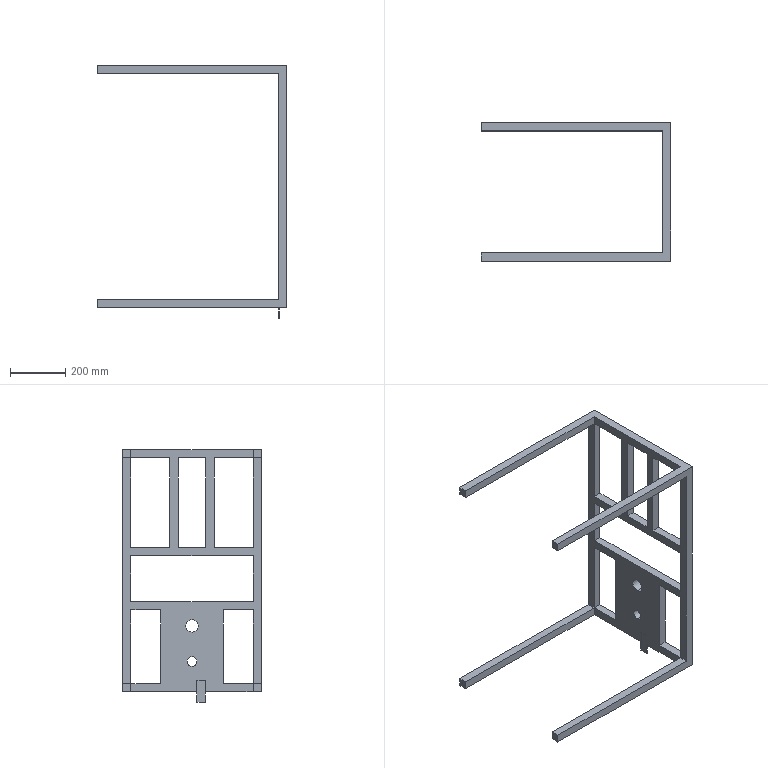Component | SolidWorks | Frame-1 | 1 solid | 55 faces | volume 7844328 mm3 | plane 51 | cylinder 4 | commonest cylinder face diameters 46 x2 35 x2